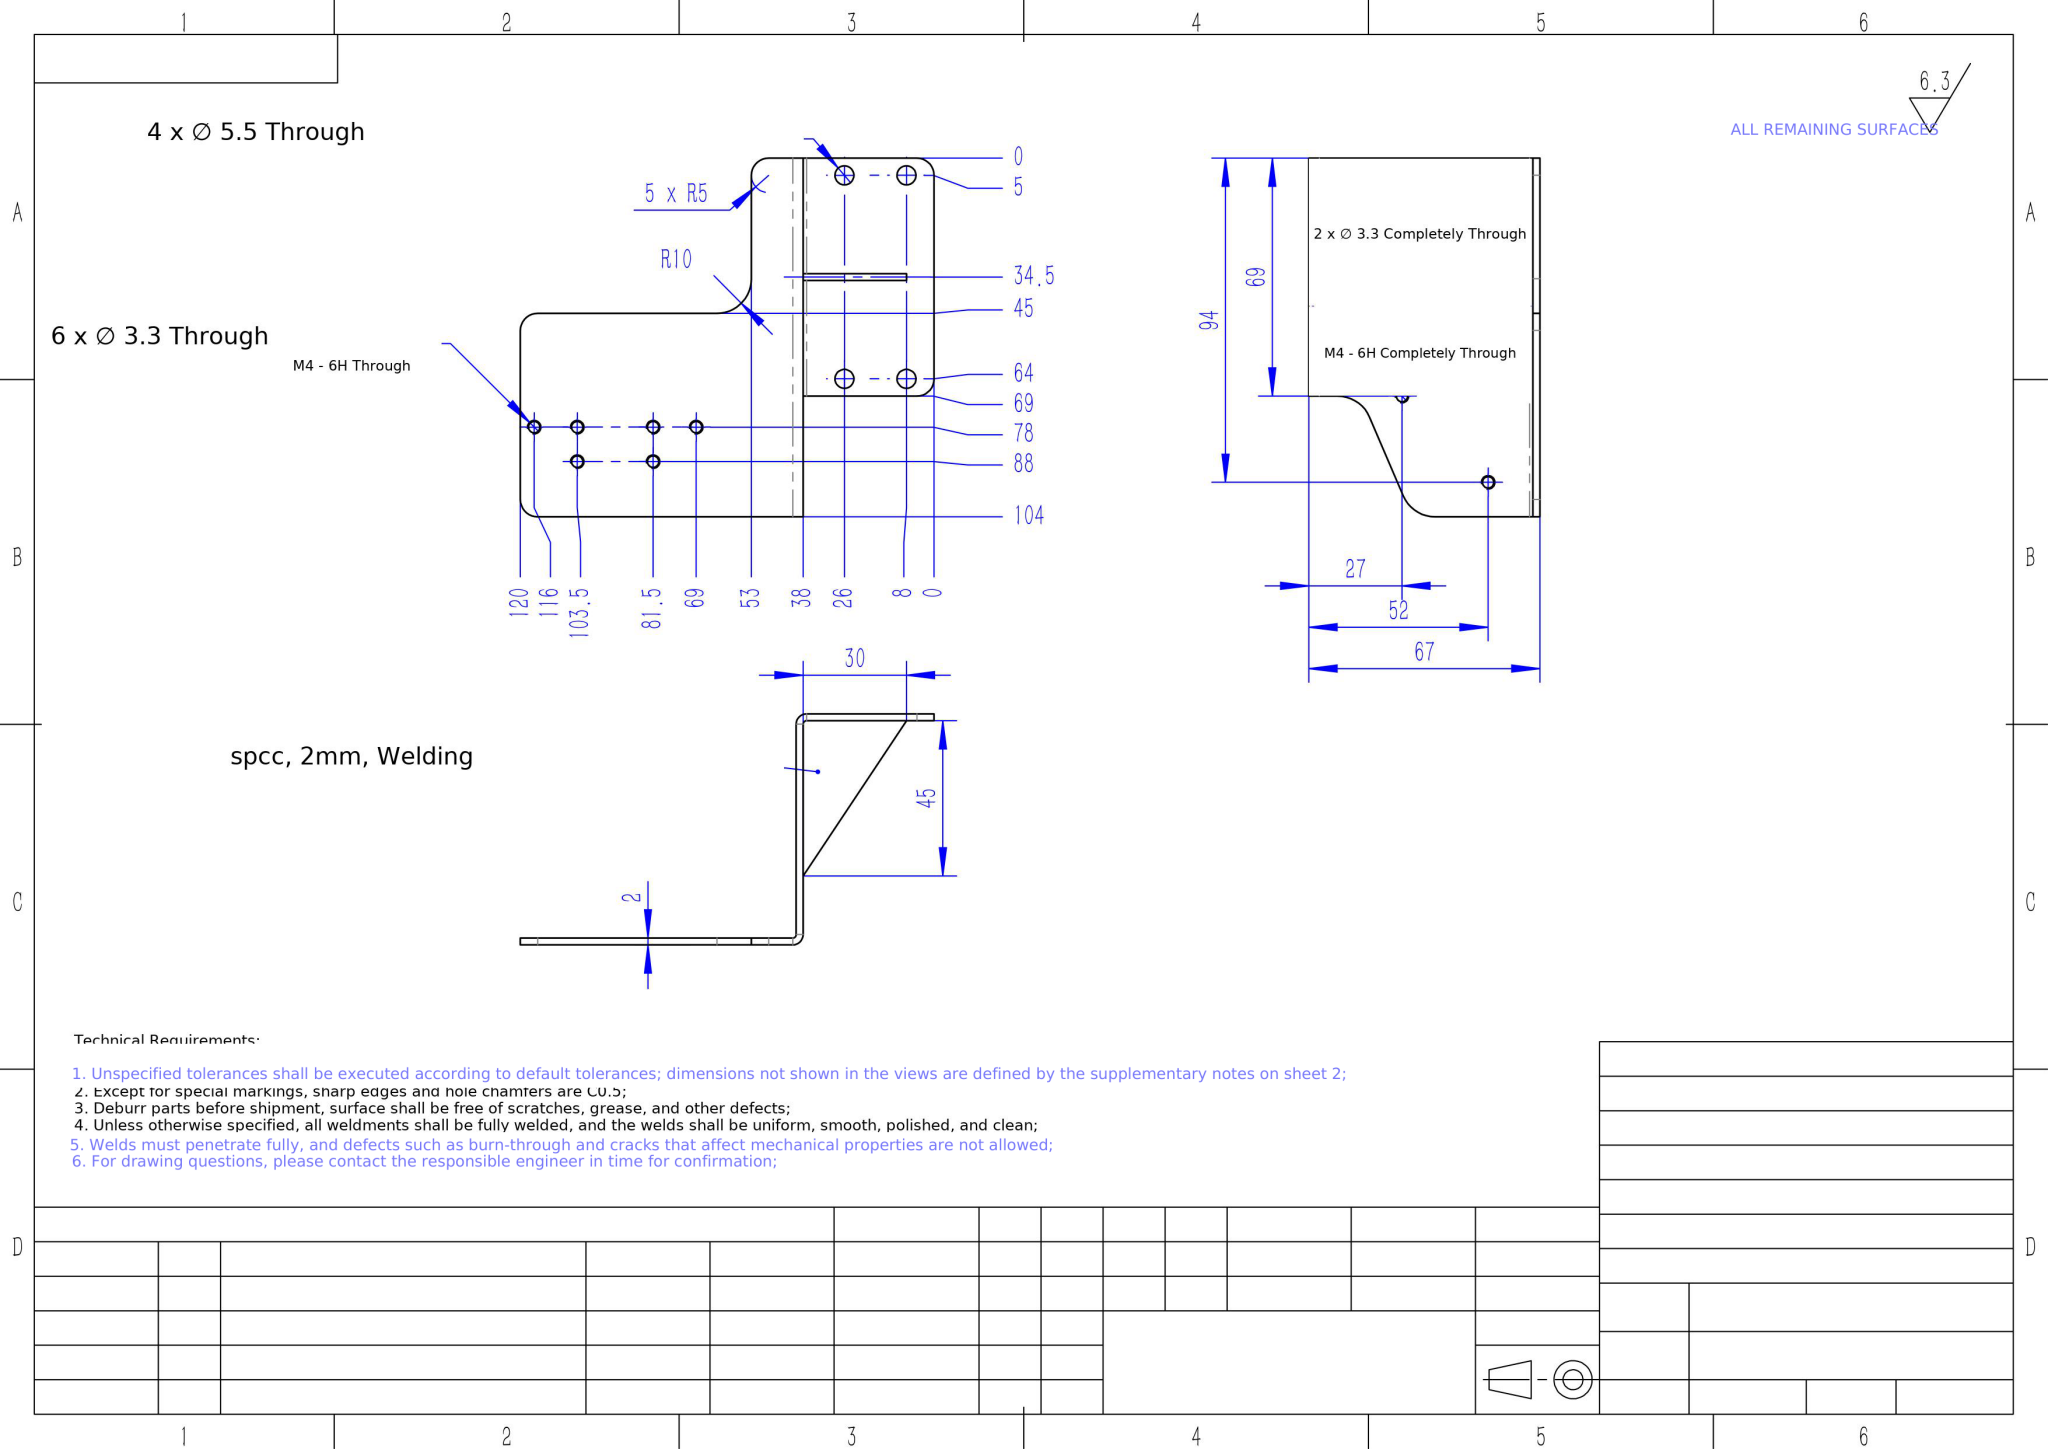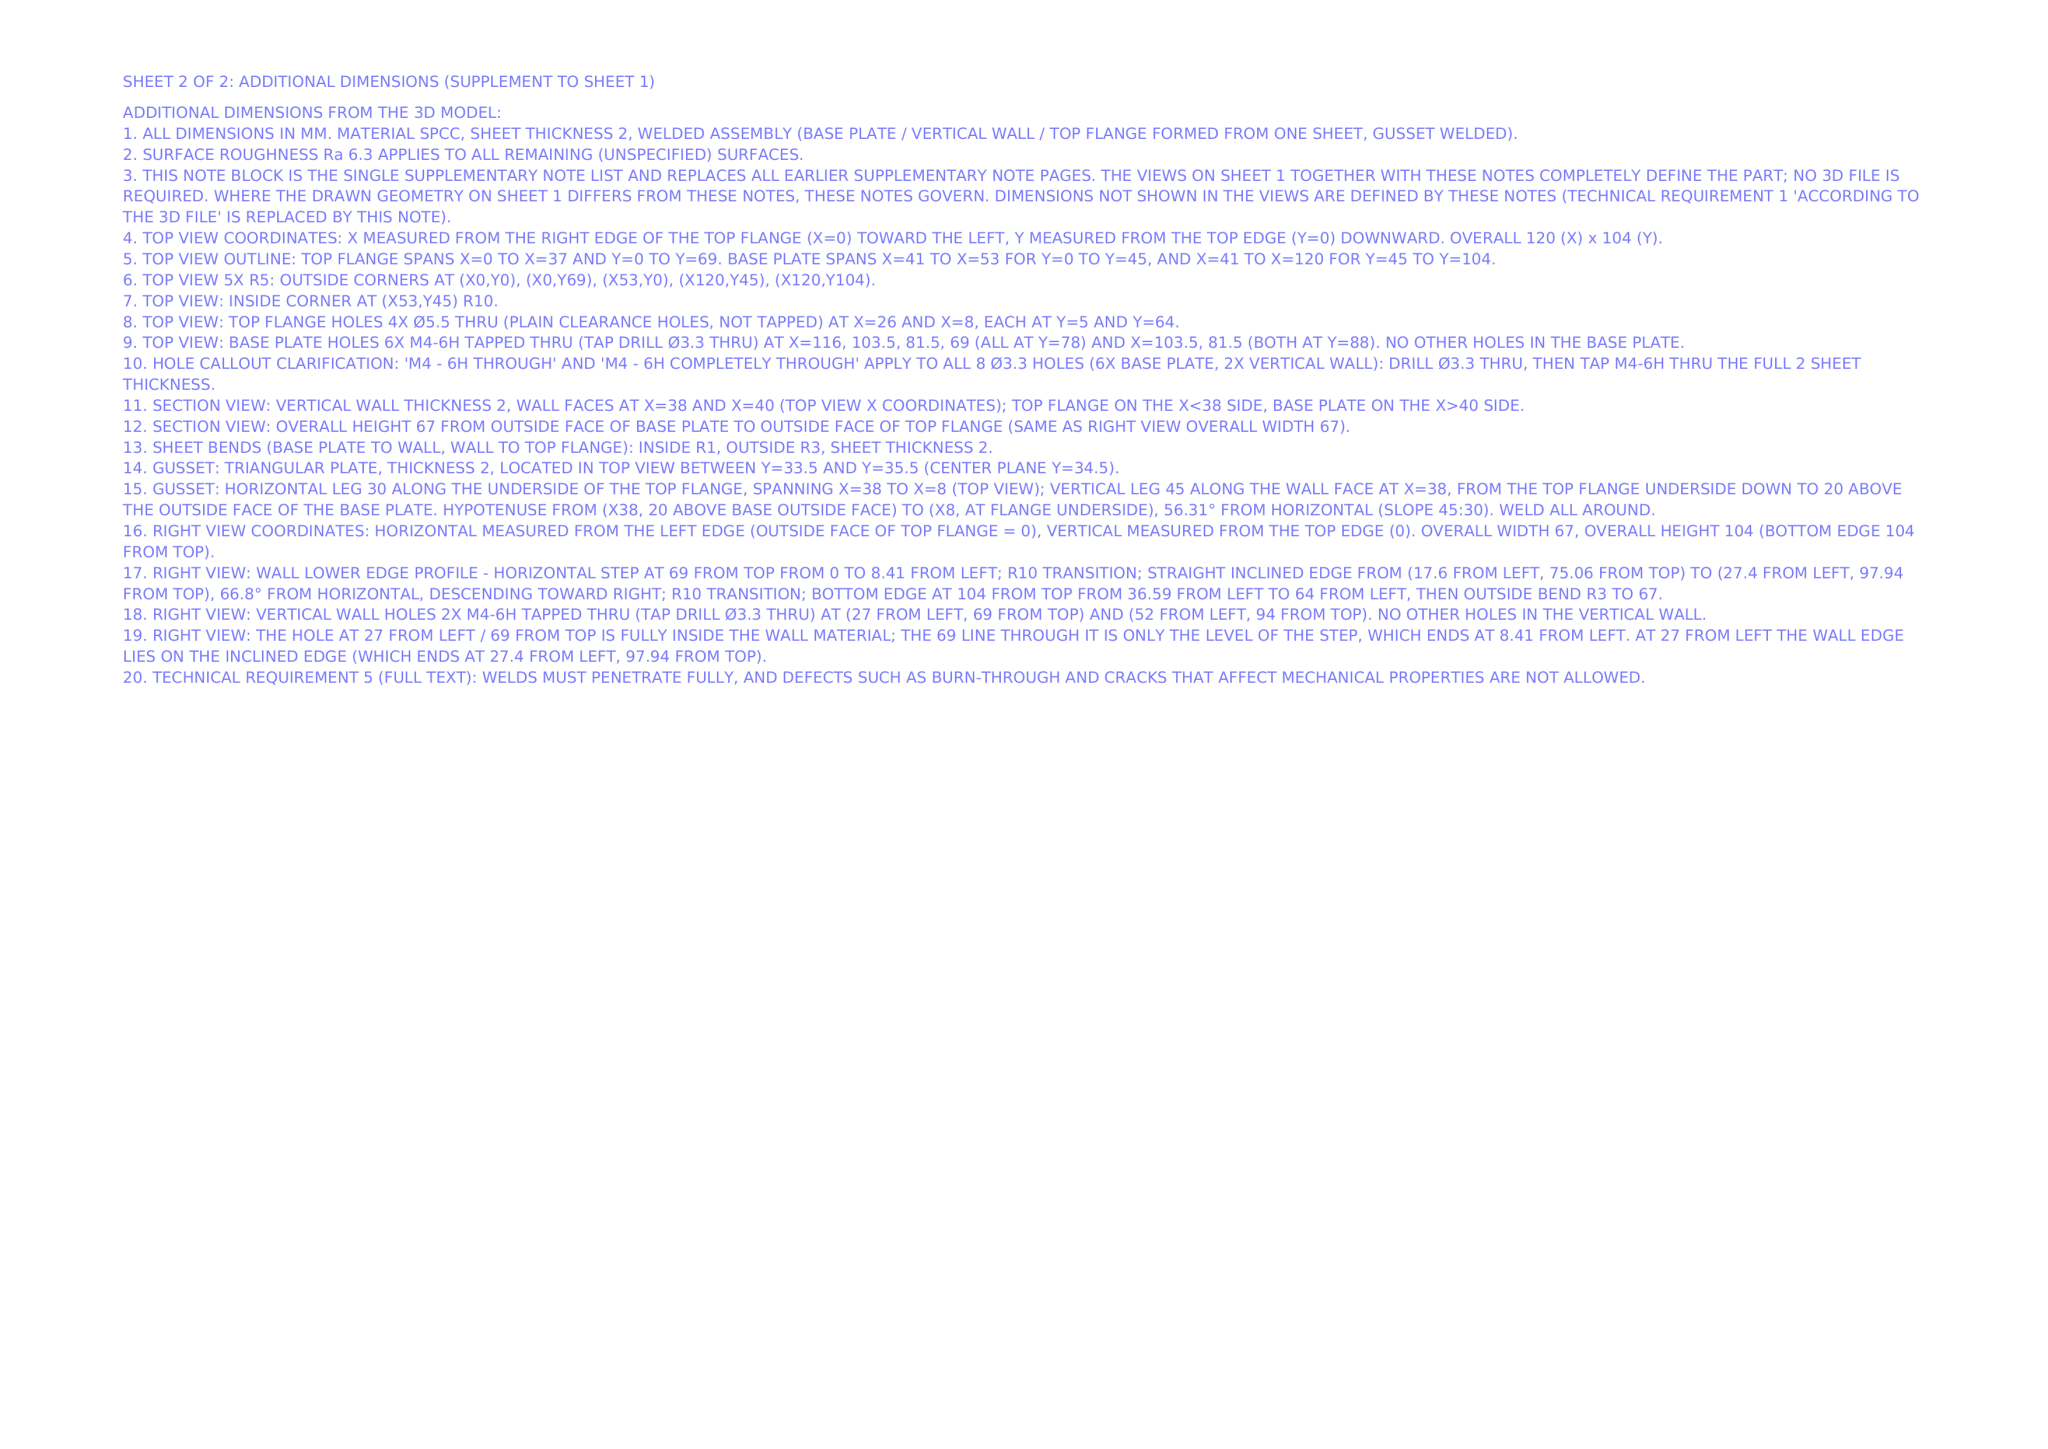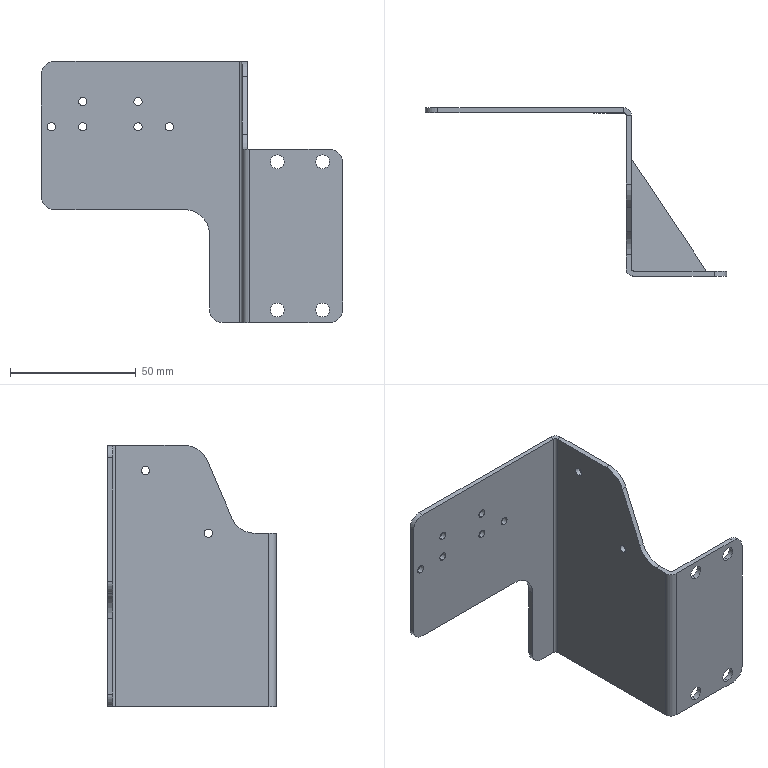Part | NX | mm | 1 solid | 60 faces | box 120 x 67 x 104 mm | volume 28930 mm3 | cylinder 37 | plane 23 | commonest cylinder face diameters 3.3 x16 5.5 x8 10 x5 2 x3 20 x3 6 x2